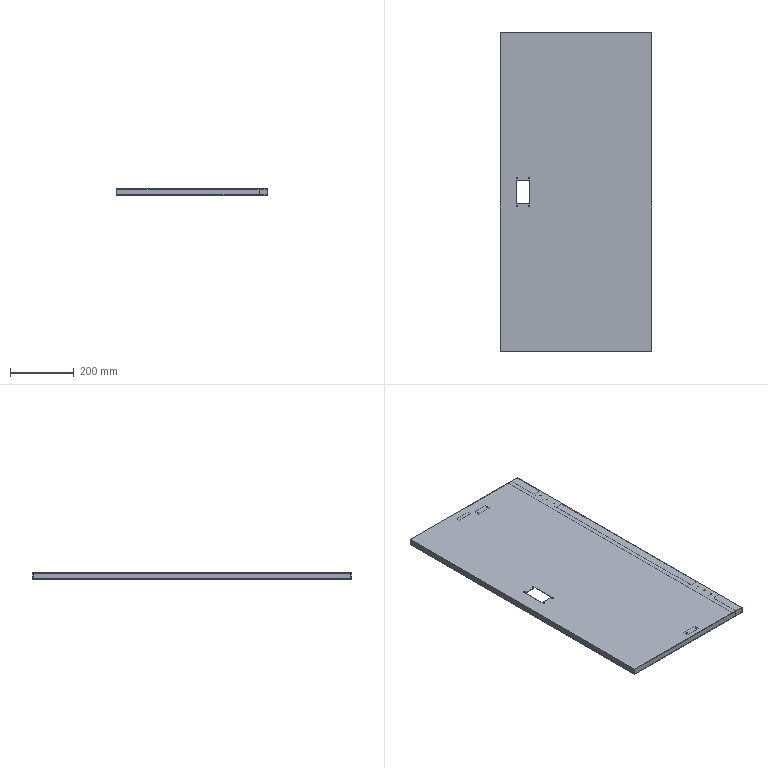Component | SolidWorks | SYM0671-81-300-1_SYM0671-81-301-1 | 1 solid | 106 faces | box 474 x 996 x 20 mm | volume 953851 mm3 | plane 74 | cylinder 32 | commonest cylinder face diameters 3 x12 4 x12 5 x8 | material Steel
build123d program:
from build123d import *

# Parameters (mm, degrees)
SKETCH_1_W                      = 474
SKETCH_1_H                      = 996
EXTRUDE1_DEPTH                  = 20
SHELL_1_T                       = 1.5
CUT_EXTRUDE1_REACH              = 1105.219
SKETCH_2_W                      = 434.5
SKETCH_2_H                      = 970
SKETCH_6_W                      = 42
SKETCH_6_H                      = 73
CUT_EXTRUDE4_DEPTH              = 1104.219
SKETCH_7_W                      = 50
SKETCH_7_H                      = 17
EXTRUDE2_DEPTH                  = 5
SKETCH_8_R                      = 1.5
CUT_EXTRUDE5_DEPTH              = 6
LINEAR_PATTERN1_COUNT           = 2
LINEAR_PATTERN1_PITCH           = 40
LINEAR_PATTERN2_COUNT           = 2
LINEAR_PATTERN2_PITCH           = 925.5
LINEAR_PATTERN2_COPY_1_SKETCH_R = 1.5
LINEAR_PATTERN2_COPY_1_DEPTH    = 6
SKETCH_10_W                     = 26.5
SKETCH_10_H                     = 84
CUT_EXTRUDE6_DEPTH              = 10
LINEAR_PATTERN3_COUNT           = 2
LINEAR_PATTERN3_PITCH           = 696
SKETCH_11_W                     = 24
SKETCH_11_H                     = 100
EXTRUDE4_DEPTH                  = 9.8
EXTRUDE4_2_DEPTH                = 9.8
SKETCH_12_R                     = 2.5
CUT_EXTRUDE7_DEPTH              = 1.5
LINEAR_PATTERN4_COUNT           = 2
LINEAR_PATTERN4_PITCH           = 88
LINEAR_PATTERN4_COUNT_DIR2      = 2
LINEAR_PATTERN4_PITCH_DIR2      = 38
SKETCH_13_R                     = 2
CUT_EXTRUDE8_DEPTH              = 9.8
LINEAR_PATTERN5_COUNT           = 3
LINEAR_PATTERN5_PITCH           = 30
SKETCH_14_R                     = 2
CUT_EXTRUDE9_DEPTH              = 11.3
LINEAR_PATTERN7_COUNT           = 3
LINEAR_PATTERN7_PITCH           = 30
EXTRUDE1_2_REACH                = 1105.219
SKETCH2_W                       = 50
SKETCH2_H                       = 10
EXTRUDE2_2_DEPTH                = 15
SKETCH3_R                       = 1.5
EXTRUDE3_DEPTH                  = 6
LPATTERN1_COUNT                 = 2
LPATTERN1_PITCH                 = 40


with BuildPart() as part:
    # Sketch 1 → Extrude1 (new body)
    with BuildSketch(Plane.XY):
        with Locations((-237, 498)):
            Rectangle(SKETCH_1_W, SKETCH_1_H)
    extrude(amount=-EXTRUDE1_DEPTH)

    # Shell 1 (no face opened: a closed hollow body)
    add(offset(amount=-SHELL_1_T, mode=Mode.PRIVATE), mode=Mode.SUBTRACT)

    # Sketch 2 → Cut - Extrude1 (cut, up to next)
    with BuildSketch(Plane(origin=(0, 0, -20), x_dir=(-1, 0, 0), z_dir=(0, 0, -1)), mode=Mode.PRIVATE) as cut_extrude1_sk1:
        with Locations((243.75, 498)):
            Rectangle(SKETCH_2_W, SKETCH_2_H)
    cut_extrude1_tool1 = extrude(cut_extrude1_sk1.sketch, amount=-CUT_EXTRUDE1_REACH, mode=Mode.PRIVATE) & part.part
    add(cut_extrude1_tool1.solids().sort_by_distance((-243.75, 498, -20))[0], mode=Mode.SUBTRACT)

    # Sketch 6 → Cut-Extrude4 (cut, through all)
    with BuildSketch(Plane.XY):
        with Locations((-403, 498)):
            Rectangle(SKETCH_6_W, SKETCH_6_H)
    extrude(amount=-CUT_EXTRUDE4_DEPTH, mode=Mode.SUBTRACT)

    # Sketch 7 → Extrude2 (add)
    with BuildSketch(Plane(origin=(0, 0, -1.5), x_dir=(-1, 0, 0), z_dir=(0, 0, -1))):
        with Locations((200, 24.5)):
            Rectangle(SKETCH_7_W, SKETCH_7_H)
    extrude2 = extrude(amount=EXTRUDE2_DEPTH)

    # Sketch 8 → Cut-Extrude5 (cut)
    with BuildSketch(Plane(origin=(0, 0, -6.5), x_dir=(-1, 0, 0), z_dir=(0, 0, -1))):
        with Locations((180, 24.5)):
            Circle(SKETCH_8_R)
    cut_extrude5 = extrude(amount=-CUT_EXTRUDE5_DEPTH, mode=Mode.SUBTRACT)

    # Linear Pattern1: Cut-Extrude5 ×2
    with Locations(*[(-i * LINEAR_PATTERN1_PITCH, 0, 0) for i in range(1, LINEAR_PATTERN1_COUNT)]):
        add(cut_extrude5, mode=Mode.SUBTRACT)

    # Linear Pattern2: Extrude2, Cut-Extrude5 ×2
    with Locations(*[(0, i * LINEAR_PATTERN2_PITCH, 0) for i in range(1, LINEAR_PATTERN2_COUNT)]):
        add(extrude2)
        add(cut_extrude5, mode=Mode.SUBTRACT)

    # Linear Pattern2 copy 1 sketch → Linear Pattern2 copy 1 (cut)
    with BuildSketch(Plane(origin=(-40, 925.5, -6.5), x_dir=(-1, 0, 0), z_dir=(0, 0, -1))):
        with Locations((180, 24.5)):
            Circle(LINEAR_PATTERN2_COPY_1_SKETCH_R)
    extrude(amount=-LINEAR_PATTERN2_COPY_1_DEPTH, mode=Mode.SUBTRACT)

    # Sketch 10 → Cut - Extrude6 (cut)
    with BuildSketch(Plane(origin=(0, 0, -20), x_dir=(-1, 0, 0), z_dir=(0, 0, -1))):
        with Locations((13.25, 150)):
            Rectangle(SKETCH_10_W, SKETCH_10_H)
    cut_extrude6 = extrude(amount=-CUT_EXTRUDE6_DEPTH, mode=Mode.SUBTRACT)

    # Linear Pattern3: Cut - Extrude6 ×2
    with Locations(*[(0, i * LINEAR_PATTERN3_PITCH, 0) for i in range(1, LINEAR_PATTERN3_COUNT)]):
        add(cut_extrude6, mode=Mode.SUBTRACT)

    # Sketch 12 → Cut-Extrude7 (cut)
    with BuildSketch(Plane(origin=(0, 0, -1.5), x_dir=(-1, 0, 0), z_dir=(0, 0, -1))):
        with Locations((422, 542)):
            Circle(SKETCH_12_R)
    cut_extrude7 = extrude(amount=-CUT_EXTRUDE7_DEPTH, mode=Mode.SUBTRACT)

    # Linear Pattern4: Cut-Extrude7 2 × 2
    with Locations(*[(j * LINEAR_PATTERN4_PITCH_DIR2, -i * LINEAR_PATTERN4_PITCH, 0) for i in range(LINEAR_PATTERN4_COUNT) for j in range(LINEAR_PATTERN4_COUNT_DIR2) if (i, j) != (0, 0)]):
        add(cut_extrude7, mode=Mode.SUBTRACT)

    # Extrude1_2: up to this face of the body (flat: up to its plane)
    extrude1_2_end = Plane(part.part.faces().sort_by_distance((-237, 996, -10))[0])
    # Sketch1 → Extrude1_2 (add, up to the picked face)
    with BuildSketch(Plane(origin=(0, 0, 0), x_dir=(1, 0, 0), z_dir=(0, 1, 0)), mode=Mode.PRIVATE) as extrude1_2_sk1:
        Polygon((-25.5, 1.5), (-40.5, 1.5), (-40.5, 3), (-27, 3), (-27, 20), (-25.5, 20), align=None)
    extrude1_2_tool1 = split(extrude(extrude1_2_sk1.sketch, amount=EXTRUDE1_2_REACH, mode=Mode.PRIVATE), bisect_by=extrude1_2_end, keep=Keep.BOTH, mode=Mode.PRIVATE)


with BuildPart() as body_2:
    # Sketch 11 → Extrude4 (new body)
    with BuildSketch(Plane(origin=(0, 0, -1.5), x_dir=(-1, 0, 0), z_dir=(0, 0, -1))):
        with Locations((13.5, 150)):
            Rectangle(SKETCH_11_W, SKETCH_11_H)
    extrude(amount=EXTRUDE4_DEPTH)

    # Sketch 13 → Cut-Extrude8 (cut)
    with BuildSketch(Plane(origin=(0, 0, -11.3), x_dir=(-1, 0, 0), z_dir=(0, 0, -1))):
        with Locations((16, 120)):
            Circle(SKETCH_13_R)
    cut_extrude8 = extrude(amount=-CUT_EXTRUDE8_DEPTH, mode=Mode.SUBTRACT)

    # Linear Pattern5: Cut-Extrude8 ×3
    with Locations(*[(0, i * LINEAR_PATTERN5_PITCH, 0) for i in range(1, LINEAR_PATTERN5_COUNT)]):
        add(cut_extrude8, mode=Mode.SUBTRACT)


with BuildPart() as body_3:
    # Sketch 11 → Extrude4 2 (new body)
    with BuildSketch(Plane(origin=(0, 0, -1.5), x_dir=(-1, 0, 0), z_dir=(0, 0, -1))):
        with Locations((13.5, 846)):
            Rectangle(SKETCH_11_W, SKETCH_11_H)
    extrude(amount=EXTRUDE4_2_DEPTH)

    # Sketch 14 → Cut - Extrude9 (cut)
    with BuildSketch(Plane(origin=(0, 0, -11.3), x_dir=(-1, 0, 0), z_dir=(0, 0, -1))):
        with Locations((16, 816)):
            Circle(SKETCH_14_R)
    cut_extrude9 = extrude(amount=-CUT_EXTRUDE9_DEPTH, mode=Mode.SUBTRACT)

    # Linear Pattern7: Cut - Extrude9 ×3
    with Locations(*[(0, i * LINEAR_PATTERN7_PITCH, 0) for i in range(1, LINEAR_PATTERN7_COUNT)]):
        add(cut_extrude9, mode=Mode.SUBTRACT)


with BuildPart() as part_1:
    add(part.part)

    add(body_2.part)  # Extrude1_2 merges body 2

    add(body_3.part)  # Extrude1_2 merges body 3
    add(extrude1_2_tool1.solids().sort_by(Axis((-33, 0, -1.738), (0, 1, 0)))[0])

    # Sketch2 → Extrude2_2 (add)
    with BuildSketch(Plane(origin=(0, 0, -1.5), x_dir=(-1, 0, 0), z_dir=(0, 0, -1))):
        with Locations((266, 967)):
            Rectangle(SKETCH2_W, SKETCH2_H)
    extrude(amount=EXTRUDE2_2_DEPTH)

    # Sketch3 → Extrude3 (cut)
    with BuildSketch(Plane(origin=(0, 0, -16.5), x_dir=(-1, 0, 0), z_dir=(0, 0, -1))):
        with Locations((286, 967)):
            Circle(SKETCH3_R)
    extrude3 = extrude(amount=-EXTRUDE3_DEPTH, mode=Mode.SUBTRACT)

    # LPattern1: Extrude3 ×2
    with Locations(*[(i * LPATTERN1_PITCH, 0, 0) for i in range(1, LPATTERN1_COUNT)]):
        add(extrude3, mode=Mode.SUBTRACT)


solid = part_1.part

# Placed as in the assembly
solid = solid.moved(Location((547.251, -512.857, 1051.018), (0, 0, 0)))